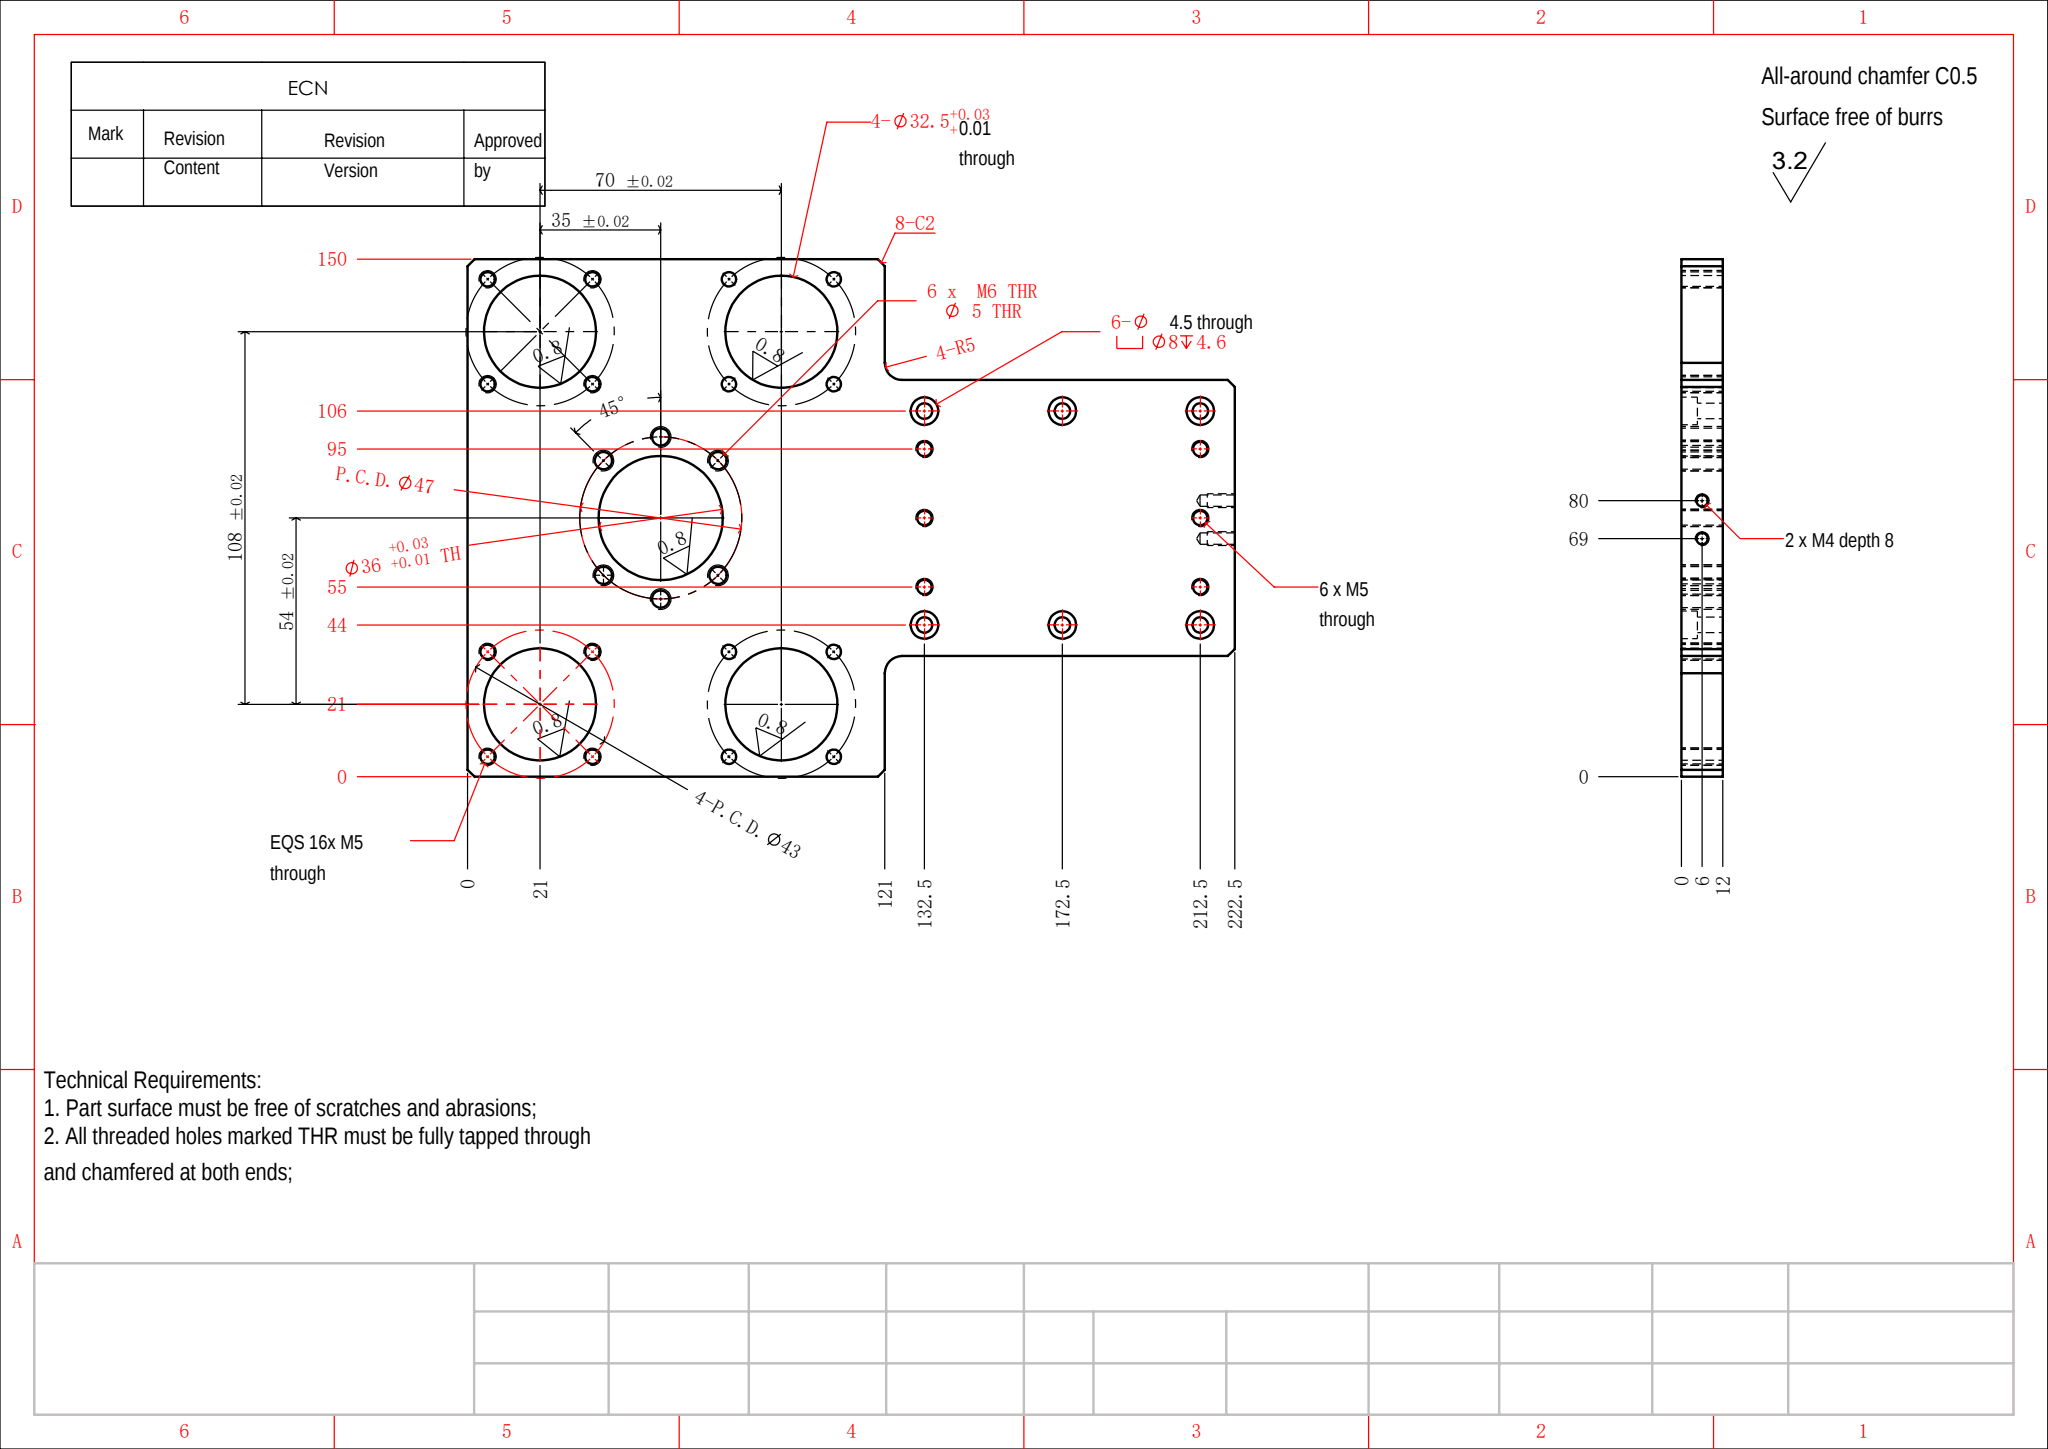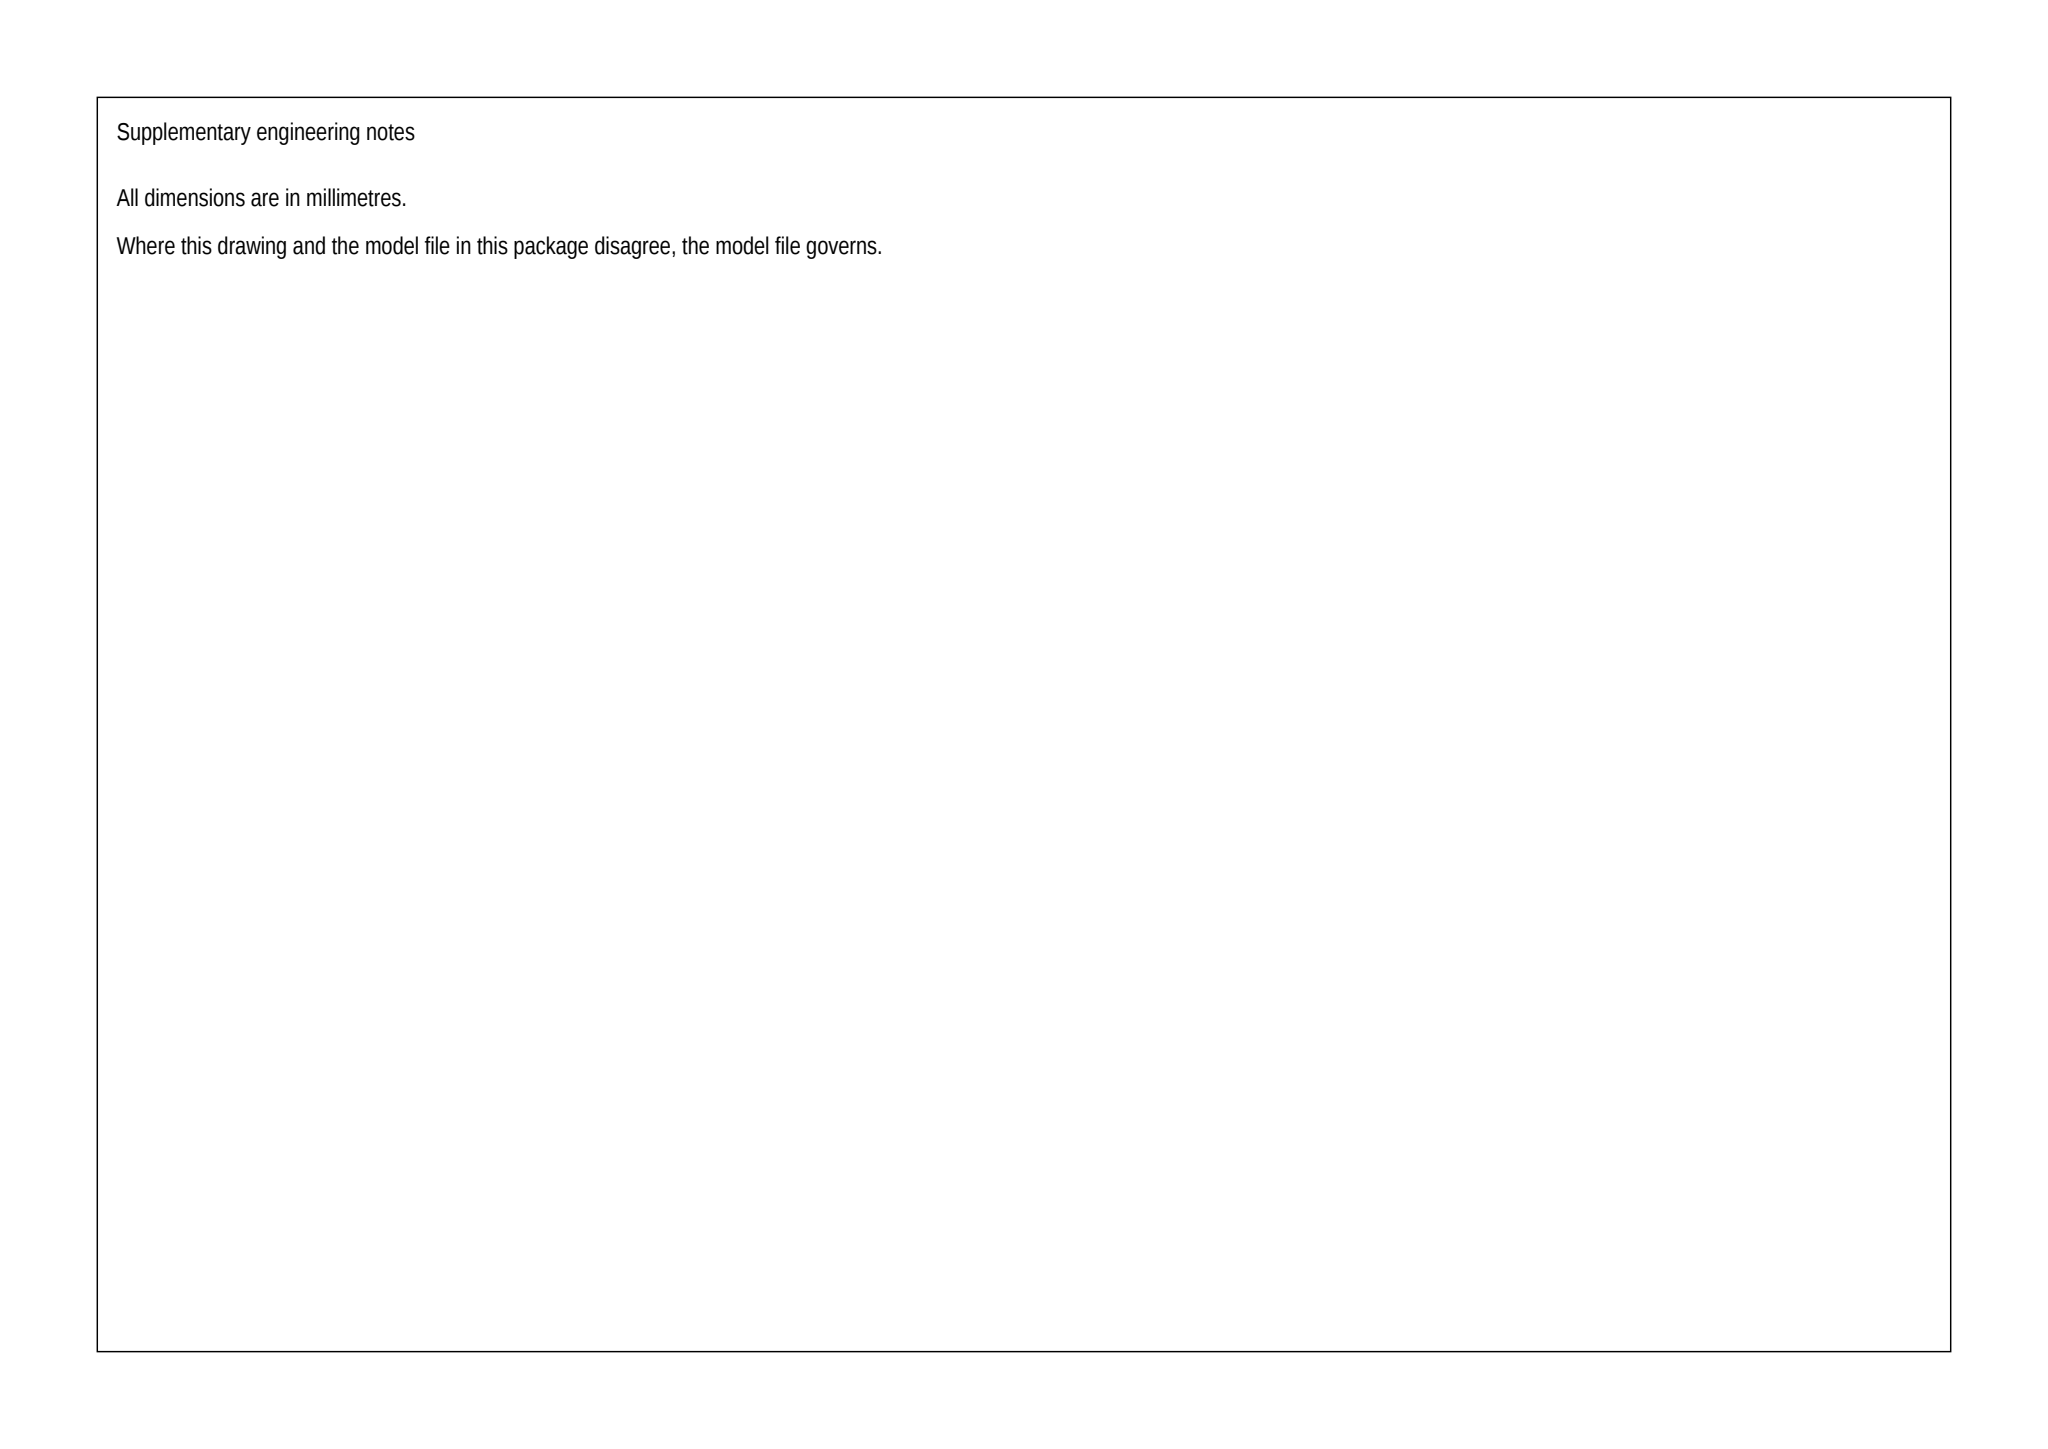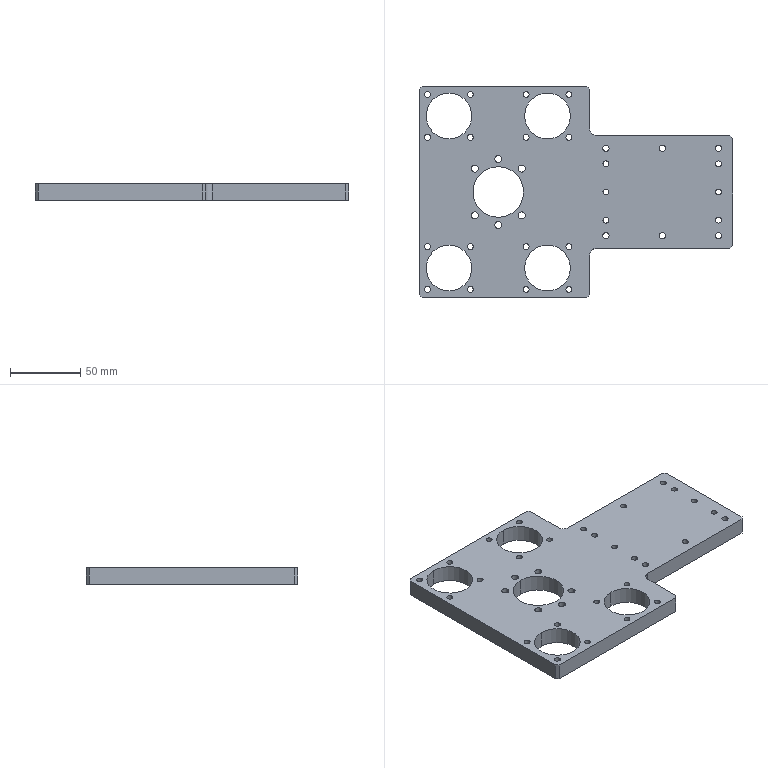Part | SolidWorks | mm | 1 solid | 122 faces | box 222.5 x 150 x 12 mm | volume 255847 mm3 | cylinder 96 | plane 22 | cone 4 | commonest cylinder face diameters 4.2 x44 5 x12 4.5 x12 8 x12 32.5 x8 3.3 x4 36 x2 10 x2
Drawing notes:
OVERALL 222.5 x 150 x 12 THK | from the solid: bbox_xyz 222.5 x 150.0 x 12.0
STEP CUT X121 TO X222.5: 80 WIDE, Y35 TO Y115 FROM BTM EDGE | from the solid: axis_planes x=121 (2), x=222.5, y=35, y=115 define L-shaped step; bbox 222.5 x 150
6 x M5 THRU 12 AT X132.5 & X212.5, Y55/75/95 FROM MIN CORNER | from the solid: cylinders dia 4.2 z-axis at (132.5,55/75/95) and (212.5,55/75/95), length 12 = full thk
2 x M4 DP 8 IN RH END FACE X222.5, AT Y70 & Y81, Z6 MID-THK | from the solid: cylinders [3.3,'x',[null,70.0,6.0],10.1] and [3.3,'x',[null,81.0,6.0],10.1] + 118 deg drill cones